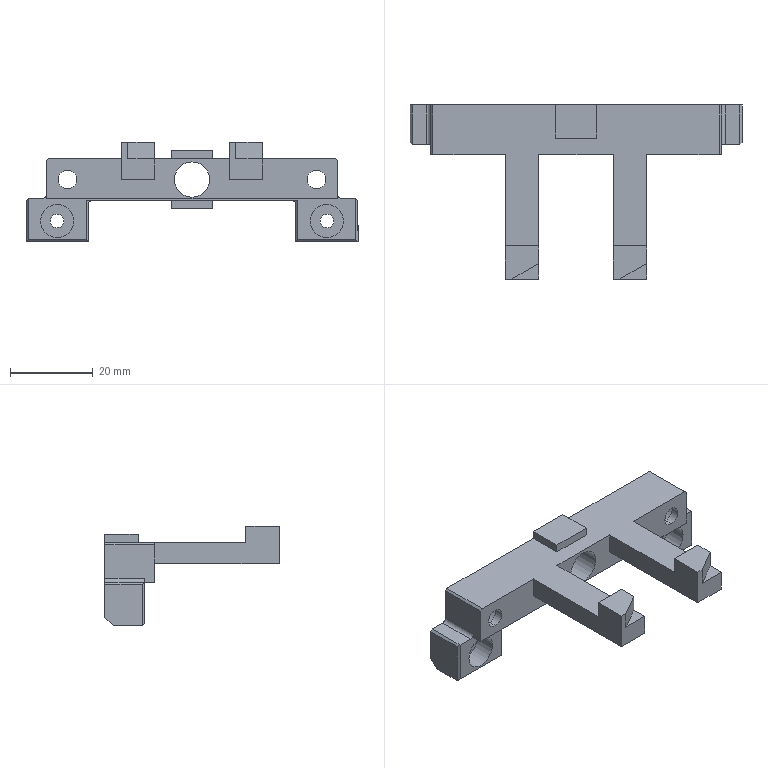Component | SolidWorks | SideMovingBlock-1 | 1 solid | 78 faces | box 80 x 42 x 24 mm | volume 11949 mm3 | plane 56 | cylinder 22 | commonest cylinder face diameters 8 x8 4.5 x4 3.3 x4 2 x4 8.5 x2
build123d program:
from build123d import *

# Parameters (mm, degrees)
SKETCH1_W             = 12
SKETCH1_H             = 70
EXTRUDE1_DEPTH        = 5
SKETCH2_W             = 5
SKETCH2_H             = 8
EXTRUDE2_DEPTH        = 30
SKETCH3_W             = 8
SKETCH3_H             = 8
EXTRUDE3_DEPTH        = 4
EXTRUDE4_DEPTH        = 4
LINEAR_PATTERN1_COUNT = 2
LINEAR_PATTERN1_PITCH = 26
SKETCH5_W             = 12
SKETCH5_H             = 70
EXTRUDE5_DEPTH        = 4.5
SKETCH8_W             = 9.5
SKETCH8_H             = 80
EXTRUDE7_DEPTH        = 10.5
SKETCH9_W             = 9.5
SKETCH9_H             = 50
EXTRUDE8_DEPTH        = 10
CHAMFER1_SIZE         = 0.5
CHAMFER2_SIZE         = 2
SKETCH13_R            = 4
EXTRUDE12_DEPTH       = 10
SKETCH14_R            = 2.25
EXTRUDE13_DEPTH       = 10
SKETCH15_R            = 4.25
EXTRUDE14_DEPTH       = 60.908
FILLET1_R             = 1
FILLET2_R             = 1
SKETCH16_W            = 2
SKETCH16_H            = 10
EXTRUDE15_DEPTH       = 8
M4_TAPPED_HOLE1_D     = 3.3
SKETCH19_R            = 4
EXTRUDE16_DEPTH       = 5


with BuildPart() as part:
    # Sketch1 → Extrude1 (new body)
    with BuildSketch(Plane.XY):
        Rectangle(SKETCH1_W, SKETCH1_H)
    extrude(amount=EXTRUDE1_DEPTH)

    # Sketch2 → Extrude2 (add)
    with BuildSketch(Plane.ZY.offset(6)):
        with Locations((2.5, -13)):
            Rectangle(SKETCH2_W, SKETCH2_H)
        with Locations((2.5, 13)):
            Rectangle(SKETCH2_W, SKETCH2_H)
    extrude(amount=EXTRUDE2_DEPTH)

    # Sketch3 → Extrude3 (add)
    with BuildSketch(Plane.XY.offset(5)):
        with Locations((-32, -13)):
            Rectangle(SKETCH3_W, SKETCH3_H)
    extrude3 = extrude(amount=EXTRUDE3_DEPTH)

    # Sketch4 → Extrude4 (cut)
    with BuildSketch(Plane.XY.offset(9)):
        Polygon((-36, -10.5), (-36, -17), (-32.247, -17), align=None)
    extrude4 = extrude(amount=-EXTRUDE4_DEPTH, mode=Mode.SUBTRACT)

    # Linear Pattern1: Extrude3, Extrude4 ×2
    with Locations(*[(0, i * LINEAR_PATTERN1_PITCH, 0) for i in range(1, LINEAR_PATTERN1_COUNT)]):
        add(extrude3)
        add(extrude4, mode=Mode.SUBTRACT)

    # Sketch5 → Extrude5 (add)
    with BuildSketch(Plane(origin=(0, 0, 0), x_dir=(-1, 0, 0), z_dir=(0, 0, -1))):
        Rectangle(SKETCH5_W, SKETCH5_H)
    extrude(amount=EXTRUDE5_DEPTH)

    # Sketch8 → Extrude7 (add)
    with BuildSketch(Plane(origin=(0, 0, -4.5), x_dir=(-1, 0, 0), z_dir=(0, 0, -1))):
        with Locations((-1.25, 0)):
            Rectangle(SKETCH8_W, SKETCH8_H)
    extrude(amount=EXTRUDE7_DEPTH)

    # Sketch9 → Extrude8 (cut)
    with BuildSketch(Plane(origin=(0, 0, -15), x_dir=(-1, 0, 0), z_dir=(0, 0, -1))):
        with Locations((-1.25, 0)):
            Rectangle(SKETCH9_W, SKETCH9_H)
    extrude(amount=-EXTRUDE8_DEPTH, mode=Mode.SUBTRACT)

    # Chamfer1
    chamfer1_edges = [part.edges().sort_by_distance(p)[0] for p in [
        (-3.5, 25, -10),
        (-3.5, 32.5, -15),
        (-3.5, 40, -9.75),
        (-3.5, -40, -9.75),
        (-3.5, -32.5, -15),
        (-3.5, -25, -10),
        (0, 35, 5),
        (0, -35, 5),
        (1.25, 40, -4.5),
        (1.25, -40, -4.5),
    ]]
    chamfer(chamfer1_edges, length=CHAMFER1_SIZE)

    # Chamfer2
    chamfer2_edges = [part.edges().sort_by_distance(p)[0] for p in [
        (6, 32.5, -15),
        (6, -32.5, -15),
    ]]
    chamfer(chamfer2_edges, length=CHAMFER2_SIZE)

    # Sketch13 → Extrude12 (cut)
    with BuildSketch(Plane(origin=(6, 0, 0), x_dir=(0, 0, -1), z_dir=(1, 0, 0))):
        with Locations((0, 30)):
            Circle(SKETCH13_R)
    extrude12 = extrude(amount=-EXTRUDE12_DEPTH, mode=Mode.SUBTRACT)

    # Sketch14 → Extrude13 (cut)
    with BuildSketch(Plane(origin=(-4, 0, 0), x_dir=(0, 0, -1), z_dir=(1, 0, 0))):
        with Locations((0, 30)):
            Circle(SKETCH14_R)
    extrude13 = extrude(amount=-EXTRUDE13_DEPTH, mode=Mode.SUBTRACT)

    # Mirror4: Extrude12, Extrude13 across plane
    add(extrude12.mirror(Plane.ZX), mode=Mode.SUBTRACT)
    add(extrude13.mirror(Plane.ZX), mode=Mode.SUBTRACT)

    # Sketch15 → Extrude14 (cut, through all)
    with BuildSketch(Plane(origin=(6, 0, 0), x_dir=(0, 0, -1), z_dir=(1, 0, 0))):
        Circle(SKETCH15_R)
    extrude(amount=-EXTRUDE14_DEPTH, mode=Mode.SUBTRACT)

    # Fillet1
    fillet1_edges = [part.edges().sort_by_distance(p)[0] for p in [
        (1.25, 35, -4.5),
        (1.25, -35, -4.5),
    ]]
    fillet(fillet1_edges, radius=FILLET1_R)

    # Fillet2
    fillet2_edges = [part.edges().sort_by_distance(p)[0] for p in [
        (1.5, -25, -5),
        (1.5, 25, -5),
    ]]
    fillet(fillet2_edges, radius=FILLET2_R)

    # Sketch16 → Extrude15 (add)
    with BuildSketch(Plane(origin=(6, 0, 0), x_dir=(0, 0, -1), z_dir=(1, 0, 0))):
        with Locations((-6, 0)):
            Rectangle(SKETCH16_W, SKETCH16_H)
    extrude15 = extrude(amount=-EXTRUDE15_DEPTH)

    # Mirror6: Extrude15 across plane
    add(extrude15.mirror(Plane.XY))

    # M4 Tapped Hole1 (through all)
    with Locations(Plane(origin=(6, 0, 0), x_dir=(0, 0, -1), z_dir=(1, 0, 0))):
        with Locations((10, 32.5), (10, -32.5)):
            Hole(M4_TAPPED_HOLE1_D / 2)

    # Sketch19 → Extrude16 (cut)
    with BuildSketch(Plane.ZY.offset(3.5)):
        with Locations(Location((-10, 32.5, 0), (0, 0, 270))):
            Circle(SKETCH19_R)
        with Locations(Location((-10, -32.5, 0), (0, 0, 270))):
            Circle(SKETCH19_R)
    extrude(amount=-EXTRUDE16_DEPTH, mode=Mode.SUBTRACT)


solid = part.part

# Placed as in the assembly
solid = solid.moved(Location((13, 46.098, 5), (0, 0, 90)))